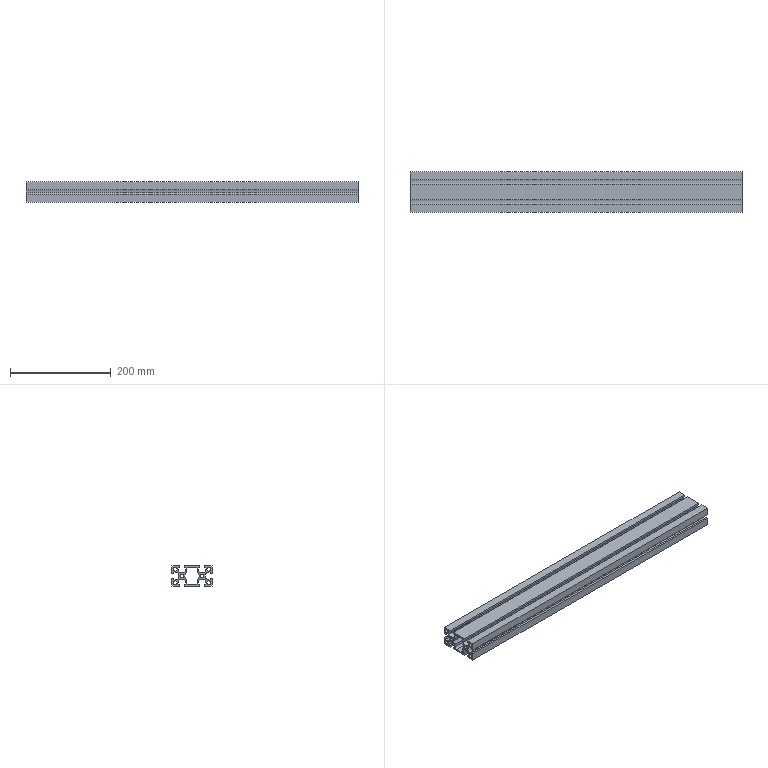Component | SolidWorks | 30-01A-1_EF4080-940-1 | 1 solid | 84 faces | box 660 x 80 x 40 mm | volume 759690 mm3 | plane 58 | cylinder 26 | commonest cylinder face diameters 8 x12 19 x10 6.8 x4
build123d program:
from build123d import *

# Parameters (mm, degrees)
SKETCH1_R      = 4
SKETCH1_R_2    = 3.4
EXTRUDE1_DEPTH = 330


with BuildPart() as part:
    # Sketch1 → Extrude1 (new, symmetric)
    with BuildSketch(Plane(origin=(0, 0, 0), x_dir=(0, 0, -1), z_dir=(1, 0, 0))):
        with BuildLine():
            Line((-40, 20), (-24.2, 20))
            Line((-24.2, 20), (-24.2, 16))
            Line((-24.2, 16), (-27.25, 16))
            Line((-27.25, 16), (-27.25, 9.361))
            ThreePointArc((-27.25, 9.361), (-20, 6), (-12.75, 9.361))
            Line((-12.75, 9.361), (-12.75, 16))
            Line((-12.75, 16), (-15.8, 16))
            Line((-15.8, 16), (-15.8, 20))
            Line((-15.8, 20), (15.8, 20))
            Line((15.8, 20), (15.8, 16))
            Line((15.8, 16), (12.75, 16))
            Line((12.75, 16), (12.75, 9.361))
            ThreePointArc((12.75, 9.361), (20, 6), (27.25, 9.361))
            Line((27.25, 9.361), (27.25, 16))
            Line((27.25, 16), (24.2, 16))
            Line((24.2, 16), (24.2, 20))
            Line((24.2, 20), (40, 20))
            Line((40, 20), (40, 4.2))
            Line((40, 4.2), (36, 4.2))
            Line((36, 4.2), (36, 7.25))
            Line((36, 7.25), (29.361, 7.25))
            ThreePointArc((29.361, 7.25), (26, 0), (29.361, -7.25))
            Line((29.361, -7.25), (36, -7.25))
            Line((36, -7.25), (36, -4.2))
            Line((36, -4.2), (40, -4.2))
            Line((40, -4.2), (40, -20))
            Line((40, -20), (24.2, -20))
            Line((24.2, -20), (24.2, -16))
            Line((24.2, -16), (27.25, -16))
            Line((27.25, -16), (27.25, -9.361))
            ThreePointArc((27.25, -9.361), (20, -6), (12.75, -9.361))
            Line((12.75, -9.361), (12.75, -16))
            Line((12.75, -16), (15.8, -16))
            Line((15.8, -16), (15.8, -20))
            Line((15.8, -20), (-15.8, -20))
            Line((-15.8, -20), (-15.8, -16))
            Line((-15.8, -16), (-12.75, -16))
            Line((-12.75, -16), (-12.75, -9.361))
            ThreePointArc((-12.75, -9.361), (-20, -6), (-27.25, -9.361))
            Line((-27.25, -9.361), (-27.25, -16))
            Line((-27.25, -16), (-24.2, -16))
            Line((-24.2, -16), (-24.2, -20))
            Line((-24.2, -20), (-40, -20))
            Line((-40, -20), (-40, -4.2))
            Line((-40, -4.2), (-36, -4.2))
            Line((-36, -4.2), (-36, -7.25))
            Line((-36, -7.25), (-29.361, -7.25))
            ThreePointArc((-29.361, -7.25), (-26, 0), (-29.361, 7.25))
            Line((-29.361, 7.25), (-36, 7.25))
            Line((-36, 7.25), (-36, 4.2))
            Line((-36, 4.2), (-40, 4.2))
            Line((-40, 4.2), (-40, 20))
        make_face()
        with Locations((-33.5, 13.5)):
            Circle(SKETCH1_R, mode=Mode.SUBTRACT)
        with Locations((-20, 0)):
            Circle(SKETCH1_R_2, mode=Mode.SUBTRACT)
        with Locations(Location((-33.5, -13.5, 0), (0, 0, 180))):
            Circle(SKETCH1_R, mode=Mode.SUBTRACT)
        with Locations((33.5, -13.5)):
            Circle(SKETCH1_R, mode=Mode.SUBTRACT)
        with Locations(Location((20, 0, 0), (0, 0, 180))):
            Circle(SKETCH1_R_2, mode=Mode.SUBTRACT)
        with Locations(Location((33.5, 13.5, 0), (0, 0, 180))):
            Circle(SKETCH1_R, mode=Mode.SUBTRACT)
        with BuildLine():
            Line((-10.5, -7.25), (-10.5, -13.5))
            ThreePointArc((-10.5, -13.5), (-9.328, -16.328), (-6.5, -17.5))
            Line((-6.5, -17.5), (6.5, -17.5))
            ThreePointArc((6.5, -17.5), (9.328, -16.328), (10.5, -13.5))
            Line((10.5, -13.5), (10.5, -7.25))
            Line((10.5, -7.25), (10.639, -7.25))
            ThreePointArc((10.639, -7.25), (14, 0), (10.639, 7.25))
            Line((10.639, 7.25), (10.5, 7.25))
            Line((10.5, 7.25), (10.5, 13.5))
            ThreePointArc((10.5, 13.5), (9.328, 16.328), (6.5, 17.5))
            Line((6.5, 17.5), (-6.5, 17.5))
            ThreePointArc((-6.5, 17.5), (-9.328, 16.328), (-10.5, 13.5))
            Line((-10.5, 13.5), (-10.5, 7.25))
            Line((-10.5, 7.25), (-10.639, 7.25))
            ThreePointArc((-10.639, 7.25), (-14, 0), (-10.639, -7.25))
            Line((-10.639, -7.25), (-10.5, -7.25))
        make_face(mode=Mode.SUBTRACT)
    extrude(amount=EXTRUDE1_DEPTH, both=True)


solid = part.part

# Placed as in the assembly
solid = solid.moved(Location((-77.43, -497.845, 20), (90, 0, 0)))